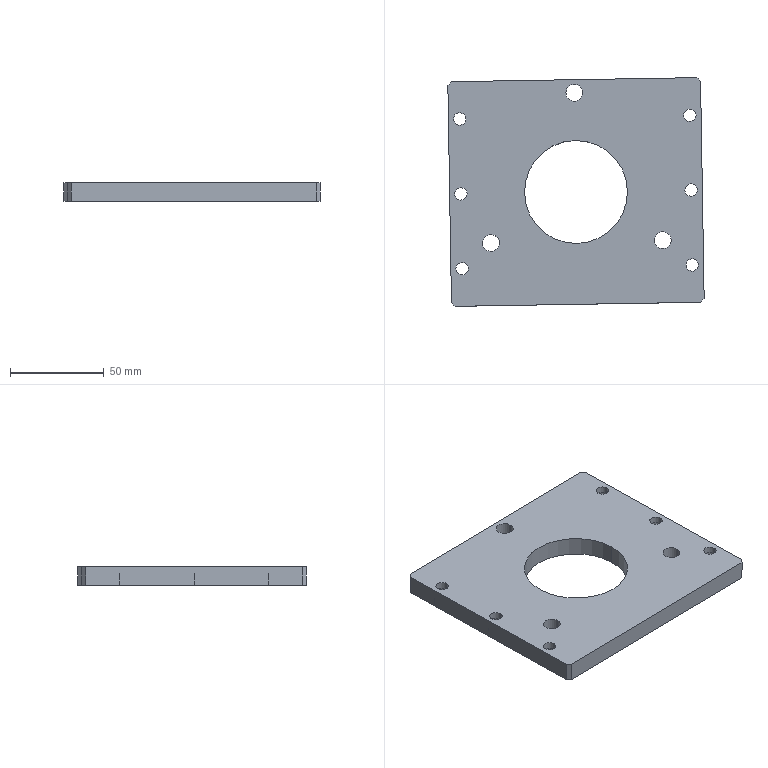Component | SolidWorks | 8TC-A17001-20-11MountingPlate-1 | 1 solid | 48 faces | box 136.89 x 122.14 x 10 mm | volume 131865 mm3 | cylinder 32 | plane 16 | commonest cylinder face diameters 11 x12 6.6 x12 9 x6 55 x2 | material A3
build123d program:
from build123d import *

# Parameters (mm, degrees)
SKETCH1_W                                       = 135
SKETCH1_H                                       = 120
SKETCH1_R                                       = 27.5
BOSS_EXTRUDE1_DEPTH                             = 10
M6_HEX_SOCKET_HEAD_CAP_SCREW_CBORE1_D           = 6.6
M6_HEX_SOCKET_HEAD_CAP_SCREW_CBORE1_DEPTH       = 12
M6_HEX_SOCKET_HEAD_CAP_SCREW_CBORE1_CBORE_D     = 11
M6_HEX_SOCKET_HEAD_CAP_SCREW_CBORE1_CBORE_DEPTH = 6.4
M6_HEX_SOCKET_HEAD_CAP_SCREW_CBORE1_TIP         = 1.983
CHAMFER1_SIZE                                   = 2
M8_CLEARANCE_HOLE1_D                            = 9
M8_CLEARANCE_HOLE1_DEPTH                        = 10
M8_CLEARANCE_HOLE1_TIP                          = 2.704


with BuildPart() as part:
    # Sketch1 → Boss-Extrude1 (new body)
    with BuildSketch(Plane.XY):
        Rectangle(SKETCH1_W, SKETCH1_H)
        Circle(SKETCH1_R, mode=Mode.SUBTRACT)
    extrude(amount=BOSS_EXTRUDE1_DEPTH)

    # M6 Hex Socket Head Cap Screw CBORE1
    with Locations(Plane(origin=(0, 0, 0), x_dir=(-1, 0, 0), z_dir=(0, 0, -1))):
        with Locations((61.5, 40), (-61.5, 40), (-61.5, 0), (61.5, 0), (-61.5, -40), (61.5, -40)):
            CounterBoreHole(M6_HEX_SOCKET_HEAD_CAP_SCREW_CBORE1_D / 2, M6_HEX_SOCKET_HEAD_CAP_SCREW_CBORE1_CBORE_D / 2, M6_HEX_SOCKET_HEAD_CAP_SCREW_CBORE1_CBORE_DEPTH, depth=M6_HEX_SOCKET_HEAD_CAP_SCREW_CBORE1_DEPTH)
            with Locations((0, 0, -(M6_HEX_SOCKET_HEAD_CAP_SCREW_CBORE1_DEPTH + M6_HEX_SOCKET_HEAD_CAP_SCREW_CBORE1_TIP / 2))):  # 118° drill point
                Cone(0, M6_HEX_SOCKET_HEAD_CAP_SCREW_CBORE1_D / 2, M6_HEX_SOCKET_HEAD_CAP_SCREW_CBORE1_TIP, mode=Mode.SUBTRACT)

    # Chamfer1
    chamfer1_edges = [part.edges().sort_by_distance(p)[0] for p in [
        (67.5, -60, 5),
        (-67.5, -60, 5),
        (-67.5, 60, 5),
        (67.5, 60, 5),
    ]]
    chamfer(chamfer1_edges, length=CHAMFER1_SIZE)

    # M8 Clearance Hole1
    with Locations(Plane.XY.offset(10)):
        with Locations((0, 53), (45.899, -26.5), (-45.899, -26.5)):
            Hole(M8_CLEARANCE_HOLE1_D / 2, depth=M8_CLEARANCE_HOLE1_DEPTH)
            with Locations((0, 0, -(M8_CLEARANCE_HOLE1_DEPTH + M8_CLEARANCE_HOLE1_TIP / 2))):  # 118° drill point
                Cone(0, M8_CLEARANCE_HOLE1_D / 2, M8_CLEARANCE_HOLE1_TIP, mode=Mode.SUBTRACT)


solid = part.part

# Placed as in the assembly
solid = solid.moved(Location((733.029, 200.722, -104.5), (0, 0, 0.9427)))